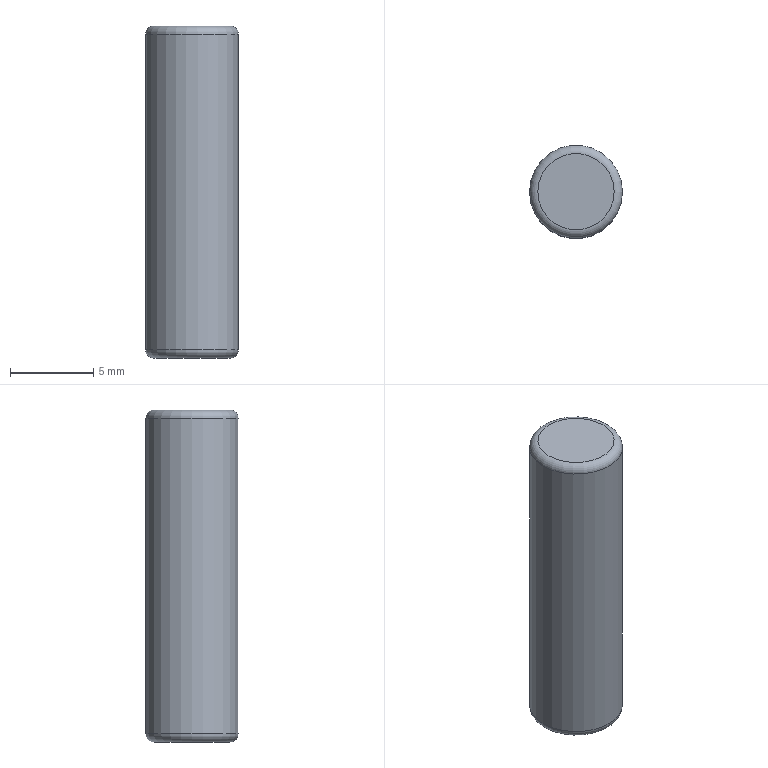Component | NX | PART_2 | 1 solid | 5 faces | box 5.6 x 5.6 x 20 mm | volume 491 mm3 | plane 2 | torus 2 | cylinder 1 | commonest cylinder face diameters 5.6 x1
STEP:
#1=CARTESIAN_POINT('',(0.,0.,0.));
#2=DIRECTION('',(0.,0.,1.));
#3=DIRECTION('',(1.,0.,0.));
#4=AXIS2_PLACEMENT_3D('',#1,#2,#3);
#5=CARTESIAN_POINT('',(32.3,0.,19.));
#6=VERTEX_POINT('',#5);
#7=CARTESIAN_POINT('',(30.,0.,19.));
#8=DIRECTION('',(0.,0.,1.));
#9=DIRECTION('',(1.,0.,0.));
#10=AXIS2_PLACEMENT_3D('',#7,#8,#9);
#11=CIRCLE('',#10,2.3);
#12=CARTESIAN_POINT('',(30.,0.,19.));
#13=DIRECTION('',(0.,0.,1.));
#14=DIRECTION('',(1.,0.,0.));
#15=AXIS2_PLACEMENT_3D('',#12,#13,#14);
#16=PLANE('',#15);
#17=CARTESIAN_POINT('',(0.,0.));
#18=DIRECTION('',(1.,0.));
#19=AXIS2_PLACEMENT_2D('',#17,#18);
#20=CIRCLE('',#19,2.3);
#21=(GEOMETRIC_REPRESENTATION_CONTEXT(2)PARAMETRIC_REPRESENTATION_CONTEXT()REPRESENTATION_CONTEXT('',''));
#22=DEFINITIONAL_REPRESENTATION('',(#20),#21);
#23=PCURVE('',#16,#22);
#24=CARTESIAN_POINT('',(30.,0.,18.5));
#25=DIRECTION('',(0.,0.,1.));
#26=DIRECTION('',(1.,0.,0.));
#27=AXIS2_PLACEMENT_3D('',#24,#25,#26);
#28=TOROIDAL_SURFACE('',#27,2.3,0.5);
#29=CARTESIAN_POINT('',(0.,7.854));
#30=DIRECTION('',(1.,0.));
#31=VECTOR('',#30,1.);
#32=LINE('',#29,#31);
#33=(GEOMETRIC_REPRESENTATION_CONTEXT(2)PARAMETRIC_REPRESENTATION_CONTEXT()REPRESENTATION_CONTEXT('',''));
#34=DEFINITIONAL_REPRESENTATION('',(#32),#33);
#35=PCURVE('',#28,#34);
#36=SURFACE_CURVE('',#11,(#23,#35),.PCURVE_S1.);
#37=EDGE_CURVE('',#6,#6,#36,.T.);
#38=ORIENTED_EDGE('',*,*,#37,.T.);
#39=EDGE_LOOP('',(#38));
#40=FACE_BOUND('',#39,.T.);
#41=ADVANCED_FACE('',(#40),#16,.T.);
#42=CARTESIAN_POINT('',(27.7,0.,-1.));
#43=VERTEX_POINT('',#42);
#44=CARTESIAN_POINT('',(30.,0.,-1.));
#45=DIRECTION('',(0.,0.,-1.));
#46=DIRECTION('',(-1.,0.,0.));
#47=AXIS2_PLACEMENT_3D('',#44,#45,#46);
#48=CIRCLE('',#47,2.3);
#49=CARTESIAN_POINT('',(30.,0.,-1.));
#50=DIRECTION('',(0.,0.,-1.));
#51=DIRECTION('',(-1.,0.,0.));
#52=AXIS2_PLACEMENT_3D('',#49,#50,#51);
#53=PLANE('',#52);
#54=CARTESIAN_POINT('',(0.,0.));
#55=DIRECTION('',(1.,0.));
#56=AXIS2_PLACEMENT_2D('',#54,#55);
#57=CIRCLE('',#56,2.3);
#58=(GEOMETRIC_REPRESENTATION_CONTEXT(2)PARAMETRIC_REPRESENTATION_CONTEXT()REPRESENTATION_CONTEXT('',''));
#59=DEFINITIONAL_REPRESENTATION('',(#57),#58);
#60=PCURVE('',#53,#59);
#61=CARTESIAN_POINT('',(30.,0.,-0.5));
#62=DIRECTION('',(0.,0.,-1.));
#63=DIRECTION('',(-1.,0.,0.));
#64=AXIS2_PLACEMENT_3D('',#61,#62,#63);
#65=TOROIDAL_SURFACE('',#64,2.3,0.5);
#66=CARTESIAN_POINT('',(0.,7.854));
#67=DIRECTION('',(1.,0.));
#68=VECTOR('',#67,1.);
#69=LINE('',#66,#68);
#70=(GEOMETRIC_REPRESENTATION_CONTEXT(2)PARAMETRIC_REPRESENTATION_CONTEXT()REPRESENTATION_CONTEXT('',''));
#71=DEFINITIONAL_REPRESENTATION('',(#69),#70);
#72=PCURVE('',#65,#71);
#73=SURFACE_CURVE('',#48,(#60,#72),.PCURVE_S1.);
#74=EDGE_CURVE('',#43,#43,#73,.T.);
#75=ORIENTED_EDGE('',*,*,#74,.T.);
#76=EDGE_LOOP('',(#75));
#77=FACE_BOUND('',#76,.T.);
#78=ADVANCED_FACE('',(#77),#53,.T.);
#79=CARTESIAN_POINT('',(27.2,0.,-0.5));
#80=VERTEX_POINT('',#79);
#81=CARTESIAN_POINT('',(32.8,-0.,-0.5));
#82=VERTEX_POINT('',#81);
#83=CARTESIAN_POINT('',(30.,0.,-0.5));
#84=DIRECTION('',(0.,0.,1.));
#85=DIRECTION('',(-1.,0.,0.));
#86=AXIS2_PLACEMENT_3D('',#83,#84,#85);
#87=CIRCLE('',#86,2.8);
#88=CARTESIAN_POINT('',(30.,0.,-1.));
#89=DIRECTION('',(0.,0.,1.));
#90=DIRECTION('',(1.,0.,0.));
#91=AXIS2_PLACEMENT_3D('',#88,#89,#90);
#92=CYLINDRICAL_SURFACE('',#91,2.8);
#93=CARTESIAN_POINT('',(3.142,0.5));
#94=DIRECTION('',(1.,0.));
#95=VECTOR('',#94,1.);
#96=LINE('',#93,#95);
#97=(GEOMETRIC_REPRESENTATION_CONTEXT(2)PARAMETRIC_REPRESENTATION_CONTEXT()REPRESENTATION_CONTEXT('',''));
#98=DEFINITIONAL_REPRESENTATION('',(#96),#97);
#99=PCURVE('',#92,#98);
#100=CARTESIAN_POINT('',(6.283,6.283));
#101=DIRECTION('',(-1.,0.));
#102=VECTOR('',#101,1.);
#103=LINE('',#100,#102);
#104=(GEOMETRIC_REPRESENTATION_CONTEXT(2)PARAMETRIC_REPRESENTATION_CONTEXT()REPRESENTATION_CONTEXT('',''));
#105=DEFINITIONAL_REPRESENTATION('',(#103),#104);
#106=PCURVE('',#65,#105);
#107=SURFACE_CURVE('',#87,(#99,#106),.PCURVE_S1.);
#108=EDGE_CURVE('',#80,#82,#107,.T.);
#109=ORIENTED_EDGE('',*,*,#108,.T.);
#110=CARTESIAN_POINT('',(32.8,0.,18.5));
#111=VERTEX_POINT('',#110);
#112=CARTESIAN_POINT('',(32.8,0.,-0.5));
#113=CARTESIAN_POINT('',(32.8,0.,18.5));
#114=B_SPLINE_CURVE_WITH_KNOTS('',1,(#112,#113),.UNSPECIFIED.,.F.,.F.,(2,2),(0.5,19.5),.PIECEWISE_BEZIER_KNOTS.);
#115=CARTESIAN_POINT('',(6.283,0.));
#116=DIRECTION('',(0.,1.));
#117=VECTOR('',#116,1.);
#118=LINE('',#115,#117);
#119=(GEOMETRIC_REPRESENTATION_CONTEXT(2)PARAMETRIC_REPRESENTATION_CONTEXT()REPRESENTATION_CONTEXT('',''));
#120=DEFINITIONAL_REPRESENTATION('',(#118),#119);
#121=PCURVE('',#92,#120);
#122=CARTESIAN_POINT('',(0.,0.));
#123=DIRECTION('',(0.,1.));
#124=VECTOR('',#123,1.);
#125=LINE('',#122,#124);
#126=(GEOMETRIC_REPRESENTATION_CONTEXT(2)PARAMETRIC_REPRESENTATION_CONTEXT()REPRESENTATION_CONTEXT('',''));
#127=DEFINITIONAL_REPRESENTATION('',(#125),#126);
#128=PCURVE('',#92,#127);
#129=SEAM_CURVE('',#114,(#121,#128),.PCURVE_S1.);
#130=EDGE_CURVE('',#82,#111,#129,.T.);
#131=ORIENTED_EDGE('',*,*,#130,.T.);
#132=CARTESIAN_POINT('',(30.,0.,18.5));
#133=DIRECTION('',(0.,0.,-1.));
#134=DIRECTION('',(1.,0.,0.));
#135=AXIS2_PLACEMENT_3D('',#132,#133,#134);
#136=CIRCLE('',#135,2.8);
#137=CARTESIAN_POINT('',(6.283,19.5));
#138=DIRECTION('',(-1.,0.));
#139=VECTOR('',#138,1.);
#140=LINE('',#137,#139);
#141=(GEOMETRIC_REPRESENTATION_CONTEXT(2)PARAMETRIC_REPRESENTATION_CONTEXT()REPRESENTATION_CONTEXT('',''));
#142=DEFINITIONAL_REPRESENTATION('',(#140),#141);
#143=PCURVE('',#92,#142);
#144=CARTESIAN_POINT('',(6.283,6.283));
#145=DIRECTION('',(-1.,0.));
#146=VECTOR('',#145,1.);
#147=LINE('',#144,#146);
#148=(GEOMETRIC_REPRESENTATION_CONTEXT(2)PARAMETRIC_REPRESENTATION_CONTEXT()REPRESENTATION_CONTEXT('',''));
#149=DEFINITIONAL_REPRESENTATION('',(#147),#148);
#150=PCURVE('',#28,#149);
#151=SURFACE_CURVE('',#136,(#143,#150),.PCURVE_S1.);
#152=EDGE_CURVE('',#111,#111,#151,.T.);
#153=ORIENTED_EDGE('',*,*,#152,.T.);
#154=ORIENTED_EDGE('',*,*,#130,.F.);
#155=CARTESIAN_POINT('',(30.,0.,-0.5));
#156=DIRECTION('',(0.,0.,1.));
#157=DIRECTION('',(-1.,0.,0.));
#158=AXIS2_PLACEMENT_3D('',#155,#156,#157);
#159=CIRCLE('',#158,2.8);
#160=CARTESIAN_POINT('',(-3.142,0.5));
#161=DIRECTION('',(1.,0.));
#162=VECTOR('',#161,1.);
#163=LINE('',#160,#162);
#164=(GEOMETRIC_REPRESENTATION_CONTEXT(2)PARAMETRIC_REPRESENTATION_CONTEXT()REPRESENTATION_CONTEXT('',''));
#165=DEFINITIONAL_REPRESENTATION('',(#163),#164);
#166=PCURVE('',#92,#165);
#167=CARTESIAN_POINT('',(6.283,6.283));
#168=DIRECTION('',(-1.,0.));
#169=VECTOR('',#168,1.);
#170=LINE('',#167,#169);
#171=(GEOMETRIC_REPRESENTATION_CONTEXT(2)PARAMETRIC_REPRESENTATION_CONTEXT()REPRESENTATION_CONTEXT('',''));
#172=DEFINITIONAL_REPRESENTATION('',(#170),#171);
#173=PCURVE('',#65,#172);
#174=SURFACE_CURVE('',#159,(#166,#173),.PCURVE_S1.);
#175=EDGE_CURVE('',#82,#80,#174,.T.);
#176=ORIENTED_EDGE('',*,*,#175,.T.);
#177=EDGE_LOOP('',(#109,#131,#153,#154,#176));
#178=FACE_BOUND('',#177,.T.);
#179=ADVANCED_FACE('',(#178),#92,.T.);
#180=ORIENTED_EDGE('',*,*,#74,.F.);
#181=CARTESIAN_POINT('',(27.2,-0.,-0.5));
#182=CARTESIAN_POINT('',(27.2,-0.,-0.6337));
#183=CARTESIAN_POINT('',(27.243,-0.,-0.7639));
#184=CARTESIAN_POINT('',(27.324,-0.,-0.876));
#185=CARTESIAN_POINT('',(27.436,-0.,-0.9575));
#186=CARTESIAN_POINT('',(27.566,-0.,-1.));
#187=CARTESIAN_POINT('',(27.7,-0.,-1.));
#188=(BOUNDED_CURVE()B_SPLINE_CURVE(6,(#181,#182,#183,#184,#185,#186,#187),.UNSPECIFIED.,.F.,.F.)B_SPLINE_CURVE_WITH_KNOTS((7,7),(0.,1.571),.PIECEWISE_BEZIER_KNOTS.)CURVE()GEOMETRIC_REPRESENTATION_ITEM()RATIONAL_B_SPLINE_CURVE((1.031,1.01,0.9979,0.994,0.9979,1.01,1.031))REPRESENTATION_ITEM(''));
#189=CARTESIAN_POINT('',(0.,6.283));
#190=DIRECTION('',(0.,1.));
#191=VECTOR('',#190,1.);
#192=LINE('',#189,#191);
#193=(GEOMETRIC_REPRESENTATION_CONTEXT(2)PARAMETRIC_REPRESENTATION_CONTEXT()REPRESENTATION_CONTEXT('',''));
#194=DEFINITIONAL_REPRESENTATION('',(#192),#193);
#195=PCURVE('',#65,#194);
#196=CARTESIAN_POINT('',(6.283,6.283));
#197=DIRECTION('',(0.,1.));
#198=VECTOR('',#197,1.);
#199=LINE('',#196,#198);
#200=(GEOMETRIC_REPRESENTATION_CONTEXT(2)PARAMETRIC_REPRESENTATION_CONTEXT()REPRESENTATION_CONTEXT('',''));
#201=DEFINITIONAL_REPRESENTATION('',(#199),#200);
#202=PCURVE('',#65,#201);
#203=SEAM_CURVE('',#188,(#195,#202),.PCURVE_S1.);
#204=EDGE_CURVE('',#80,#43,#203,.T.);
#205=ORIENTED_EDGE('',*,*,#204,.F.);
#206=ORIENTED_EDGE('',*,*,#175,.F.);
#207=ORIENTED_EDGE('',*,*,#108,.F.);
#208=ORIENTED_EDGE('',*,*,#204,.T.);
#209=EDGE_LOOP('',(#180,#205,#206,#207,#208));
#210=FACE_BOUND('',#209,.T.);
#211=ADVANCED_FACE('',(#210),#65,.T.);
#212=ORIENTED_EDGE('',*,*,#37,.F.);
#213=CARTESIAN_POINT('',(32.8,-0.,18.5));
#214=CARTESIAN_POINT('',(32.8,-0.,18.634));
#215=CARTESIAN_POINT('',(32.757,-0.,18.764));
#216=CARTESIAN_POINT('',(32.676,-0.,18.876));
#217=CARTESIAN_POINT('',(32.564,-0.,18.957));
#218=CARTESIAN_POINT('',(32.434,-0.,19.));
#219=CARTESIAN_POINT('',(32.3,-0.,19.));
#220=(BOUNDED_CURVE()B_SPLINE_CURVE(6,(#213,#214,#215,#216,#217,#218,#219),.UNSPECIFIED.,.F.,.F.)B_SPLINE_CURVE_WITH_KNOTS((7,7),(0.,1.571),.PIECEWISE_BEZIER_KNOTS.)CURVE()GEOMETRIC_REPRESENTATION_ITEM()RATIONAL_B_SPLINE_CURVE((1.031,1.01,0.9979,0.994,0.9979,1.01,1.031))REPRESENTATION_ITEM(''));
#221=CARTESIAN_POINT('',(0.,6.283));
#222=DIRECTION('',(0.,1.));
#223=VECTOR('',#222,1.);
#224=LINE('',#221,#223);
#225=(GEOMETRIC_REPRESENTATION_CONTEXT(2)PARAMETRIC_REPRESENTATION_CONTEXT()REPRESENTATION_CONTEXT('',''));
#226=DEFINITIONAL_REPRESENTATION('',(#224),#225);
#227=PCURVE('',#28,#226);
#228=CARTESIAN_POINT('',(6.283,6.283));
#229=DIRECTION('',(0.,1.));
#230=VECTOR('',#229,1.);
#231=LINE('',#228,#230);
#232=(GEOMETRIC_REPRESENTATION_CONTEXT(2)PARAMETRIC_REPRESENTATION_CONTEXT()REPRESENTATION_CONTEXT('',''));
#233=DEFINITIONAL_REPRESENTATION('',(#231),#232);
#234=PCURVE('',#28,#233);
#235=SEAM_CURVE('',#220,(#227,#234),.PCURVE_S1.);
#236=EDGE_CURVE('',#111,#6,#235,.T.);
#237=ORIENTED_EDGE('',*,*,#236,.F.);
#238=ORIENTED_EDGE('',*,*,#152,.F.);
#239=ORIENTED_EDGE('',*,*,#236,.T.);
#240=EDGE_LOOP('',(#212,#237,#238,#239));
#241=FACE_BOUND('',#240,.T.);
#242=ADVANCED_FACE('',(#241),#28,.T.);
#243=CLOSED_SHELL('',(#41,#78,#179,#211,#242));
#244=MANIFOLD_SOLID_BREP('',#243);
#245=(LENGTH_UNIT()NAMED_UNIT(*)SI_UNIT(.MILLI.,.METRE.));
#246=UNCERTAINTY_MEASURE_WITH_UNIT(LENGTH_MEASURE(0.00001),#245,'','');
#247=(NAMED_UNIT(*)PLANE_ANGLE_UNIT()SI_UNIT($,.RADIAN.));
#248=(NAMED_UNIT(*)SI_UNIT($,.STERADIAN.)SOLID_ANGLE_UNIT());
#249=(GEOMETRIC_REPRESENTATION_CONTEXT(3)GLOBAL_UNCERTAINTY_ASSIGNED_CONTEXT((#246))GLOBAL_UNIT_ASSIGNED_CONTEXT((#245,#247,#248))REPRESENTATION_CONTEXT('',''));
#250=ADVANCED_BREP_SHAPE_REPRESENTATION('',(#4,#244),#249);